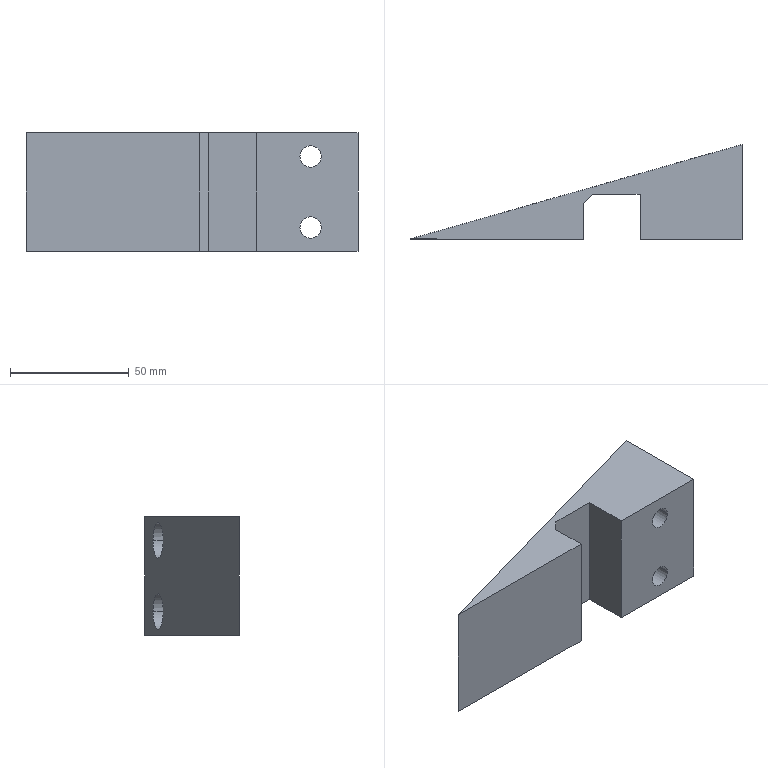Component | SolidWorks | SHYTJ-01-07-07GuideBlock-1 | 1 solid | 20 faces | box 140 x 40 x 50 mm | volume 107982 mm3 | plane 12 | cylinder 8 | commonest cylinder face diameters 15 x4 9 x4
build123d program:
from build123d import *

# Parameters (mm, degrees)
BOSS_EXTRUDE1_DEPTH                               = 50
CUT_EXTRUDE1_DEPTH                                = 154.948
HOLE_SIZE_ACCORDING_TO_TYPE_OF_SOCKET_D           = 9
HOLE_SIZE_ACCORDING_TO_TYPE_OF_SOCKET_CBORE_D     = 15
HOLE_SIZE_ACCORDING_TO_TYPE_OF_SOCKET_CBORE_DEPTH = 29


with BuildPart() as part:
    # Sketch1 → Boss-Extrude1 (new body)
    with BuildSketch(Plane.XY):
        Polygon((0, 0), (0, 40), (140, 0.149), align=None)
    extrude(amount=BOSS_EXTRUDE1_DEPTH)

    # Sketch2 → Cut-Extrude1 (cut, through all)
    with BuildSketch(Plane.XY.offset(50)):
        Polygon((43, 19.046), (63, 19.046), (67, 15.046), (67, 0.04577), (43, 0.04577), align=None)
    extrude(amount=-CUT_EXTRUDE1_DEPTH, mode=Mode.SUBTRACT)

    # Hole Size _according to_ type of socket (through all)
    with Locations(Plane(origin=(-0.04258, 40, 0), x_dir=(-1, -0.001064, 0), z_dir=(-0.001064, 1, 0))):
        with Locations((-20, 10), (-20, 40)):
            CounterBoreHole(HOLE_SIZE_ACCORDING_TO_TYPE_OF_SOCKET_D / 2, HOLE_SIZE_ACCORDING_TO_TYPE_OF_SOCKET_CBORE_D / 2, HOLE_SIZE_ACCORDING_TO_TYPE_OF_SOCKET_CBORE_DEPTH)


solid = part.part

# Placed as in the assembly
solid = solid.moved(Location((-59.116, -175.361, 293.5), (-180, 0, 180)))
STEP:
#1=COLOUR_RGB('',0.7922,0.8196,0.9333);
#2=FILL_AREA_STYLE_COLOUR('',#1);
#3=FILL_AREA_STYLE('',(#2));
#4=SURFACE_STYLE_FILL_AREA(#3);
#5=SURFACE_SIDE_STYLE('',(#4));
#6=SURFACE_STYLE_USAGE(.BOTH.,#5);
#7=PRESENTATION_STYLE_ASSIGNMENT((#6));
#8=CARTESIAN_POINT('',(-3.41,-6.47,11.161));
#9=VERTEX_POINT('',#8);
#10=CARTESIAN_POINT('',(-2.819,-6.47,11.161));
#11=VERTEX_POINT('',#10);
#12=CARTESIAN_POINT('',(-3.114,-6.47,11.161));
#13=DIRECTION('',(0.001064,1.,0.));
#14=DIRECTION('',(1.,-0.001064,0.));
#15=AXIS2_PLACEMENT_3D('',#12,#13,#14);
#16=CIRCLE('',#15,0.2953);
#17=EDGE_CURVE('',#9,#11,#16,.T.);
#18=ORIENTED_EDGE('',*,*,#17,.F.);
#19=CARTESIAN_POINT('',(-3.409,-5.637,11.161));
#20=VERTEX_POINT('',#19);
#21=CARTESIAN_POINT('',(-3.408,-5.328,11.161));
#22=DIRECTION('',(0.001064,1.,0.));
#23=VECTOR('',#22,39.37);
#24=LINE('',#21,#23);
#25=EDGE_CURVE('',#9,#20,#24,.T.);
#26=ORIENTED_EDGE('',*,*,#25,.T.);
#27=CARTESIAN_POINT('',(-2.818,-5.469,11.161));
#28=VERTEX_POINT('',#27);
#29=CARTESIAN_POINT('',(-2.818,-5.469,11.161));
#30=CARTESIAN_POINT('',(-2.818,-5.469,11.752));
#31=CARTESIAN_POINT('',(-3.409,-5.637,11.752));
#32=CARTESIAN_POINT('',(-3.409,-5.637,11.161));
#33=(BOUNDED_CURVE()B_SPLINE_CURVE(3,(#29,#30,#31,#32),.UNSPECIFIED.,.F.,.T.)B_SPLINE_CURVE_WITH_KNOTS((4,4),(0.,3.142),.UNSPECIFIED.)CURVE()GEOMETRIC_REPRESENTATION_ITEM()RATIONAL_B_SPLINE_CURVE((1.,0.3333,0.3333,1.))REPRESENTATION_ITEM(''));
#34=EDGE_CURVE('',#28,#20,#33,.T.);
#35=ORIENTED_EDGE('',*,*,#34,.F.);
#36=CARTESIAN_POINT('',(-2.818,-5.329,11.161));
#37=DIRECTION('',(0.001064,1.,0.));
#38=VECTOR('',#37,39.37);
#39=LINE('',#36,#38);
#40=EDGE_CURVE('',#11,#28,#39,.T.);
#41=ORIENTED_EDGE('',*,*,#40,.F.);
#42=EDGE_LOOP('',(#18,#26,#35,#41));
#43=FACE_OUTER_BOUND('',#42,.T.);
#44=CARTESIAN_POINT('',(-3.113,-5.328,11.161));
#45=DIRECTION('',(0.001064,1.,0.));
#46=DIRECTION('',(1.,-0.001064,0.));
#47=AXIS2_PLACEMENT_3D('',#44,#45,#46);
#48=CYLINDRICAL_SURFACE('',#47,0.2953);
#49=ADVANCED_FACE('',(#43),#48,.F.);
#50=CARTESIAN_POINT('',(-3.292,-6.903,11.161));
#51=VERTEX_POINT('',#50);
#52=CARTESIAN_POINT('',(-2.938,-6.903,11.161));
#53=VERTEX_POINT('',#52);
#54=CARTESIAN_POINT('',(-3.115,-6.903,11.161));
#55=DIRECTION('',(0.001064,1.,0.));
#56=DIRECTION('',(1.,-0.001064,0.));
#57=AXIS2_PLACEMENT_3D('',#54,#55,#56);
#58=CIRCLE('',#57,0.1772);
#59=EDGE_CURVE('',#51,#53,#58,.T.);
#60=ORIENTED_EDGE('',*,*,#59,.F.);
#61=CARTESIAN_POINT('',(-3.292,-6.47,11.161));
#62=VERTEX_POINT('',#61);
#63=CARTESIAN_POINT('',(-3.29,-5.328,11.161));
#64=DIRECTION('',(0.001064,1.,0.));
#65=VECTOR('',#64,39.37);
#66=LINE('',#63,#65);
#67=EDGE_CURVE('',#51,#62,#66,.T.);
#68=ORIENTED_EDGE('',*,*,#67,.T.);
#69=CARTESIAN_POINT('',(-2.937,-6.47,11.161));
#70=VERTEX_POINT('',#69);
#71=CARTESIAN_POINT('',(-3.114,-6.47,11.161));
#72=DIRECTION('',(0.001064,1.,0.));
#73=DIRECTION('',(1.,-0.001064,0.));
#74=AXIS2_PLACEMENT_3D('',#71,#72,#73);
#75=CIRCLE('',#74,0.1772);
#76=EDGE_CURVE('',#62,#70,#75,.T.);
#77=ORIENTED_EDGE('',*,*,#76,.T.);
#78=CARTESIAN_POINT('',(-2.936,-5.329,11.161));
#79=DIRECTION('',(0.001064,1.,0.));
#80=VECTOR('',#79,39.37);
#81=LINE('',#78,#80);
#82=EDGE_CURVE('',#53,#70,#81,.T.);
#83=ORIENTED_EDGE('',*,*,#82,.F.);
#84=EDGE_LOOP('',(#60,#68,#77,#83));
#85=FACE_OUTER_BOUND('',#84,.T.);
#86=CARTESIAN_POINT('',(-3.113,-5.328,11.161));
#87=DIRECTION('',(0.001064,1.,0.));
#88=DIRECTION('',(1.,-0.001064,0.));
#89=AXIS2_PLACEMENT_3D('',#86,#87,#88);
#90=CYLINDRICAL_SURFACE('',#89,0.1772);
#91=ADVANCED_FACE('',(#85),#90,.F.);
#92=CARTESIAN_POINT('',(-3.292,-6.903,9.98));
#93=VERTEX_POINT('',#92);
#94=CARTESIAN_POINT('',(-2.938,-6.903,9.98));
#95=VERTEX_POINT('',#94);
#96=CARTESIAN_POINT('',(-3.115,-6.903,9.98));
#97=DIRECTION('',(0.001064,1.,0.));
#98=DIRECTION('',(1.,-0.001064,0.));
#99=AXIS2_PLACEMENT_3D('',#96,#97,#98);
#100=CIRCLE('',#99,0.1772);
#101=EDGE_CURVE('',#93,#95,#100,.T.);
#102=ORIENTED_EDGE('',*,*,#101,.F.);
#103=CARTESIAN_POINT('',(-3.292,-6.47,9.98));
#104=VERTEX_POINT('',#103);
#105=CARTESIAN_POINT('',(-3.29,-5.328,9.98));
#106=DIRECTION('',(0.001064,1.,0.));
#107=VECTOR('',#106,39.37);
#108=LINE('',#105,#107);
#109=EDGE_CURVE('',#93,#104,#108,.T.);
#110=ORIENTED_EDGE('',*,*,#109,.T.);
#111=CARTESIAN_POINT('',(-2.937,-6.47,9.98));
#112=VERTEX_POINT('',#111);
#113=CARTESIAN_POINT('',(-3.114,-6.47,9.98));
#114=DIRECTION('',(0.001064,1.,0.));
#115=DIRECTION('',(1.,-0.001064,0.));
#116=AXIS2_PLACEMENT_3D('',#113,#114,#115);
#117=CIRCLE('',#116,0.1772);
#118=EDGE_CURVE('',#104,#112,#117,.T.);
#119=ORIENTED_EDGE('',*,*,#118,.T.);
#120=CARTESIAN_POINT('',(-2.936,-5.329,9.98));
#121=DIRECTION('',(0.001064,1.,0.));
#122=VECTOR('',#121,39.37);
#123=LINE('',#120,#122);
#124=EDGE_CURVE('',#95,#112,#123,.T.);
#125=ORIENTED_EDGE('',*,*,#124,.F.);
#126=EDGE_LOOP('',(#102,#110,#119,#125));
#127=FACE_OUTER_BOUND('',#126,.T.);
#128=CARTESIAN_POINT('',(-3.113,-5.328,9.98));
#129=DIRECTION('',(0.001064,1.,0.));
#130=DIRECTION('',(1.,-0.001064,0.));
#131=AXIS2_PLACEMENT_3D('',#128,#129,#130);
#132=CYLINDRICAL_SURFACE('',#131,0.1772);
#133=ADVANCED_FACE('',(#127),#132,.F.);
#134=CARTESIAN_POINT('',(-3.41,-6.47,9.98));
#135=VERTEX_POINT('',#134);
#136=CARTESIAN_POINT('',(-2.819,-6.47,9.98));
#137=VERTEX_POINT('',#136);
#138=CARTESIAN_POINT('',(-3.114,-6.47,9.98));
#139=DIRECTION('',(0.001064,1.,0.));
#140=DIRECTION('',(1.,-0.001064,0.));
#141=AXIS2_PLACEMENT_3D('',#138,#139,#140);
#142=CIRCLE('',#141,0.2953);
#143=EDGE_CURVE('',#135,#137,#142,.T.);
#144=ORIENTED_EDGE('',*,*,#143,.F.);
#145=CARTESIAN_POINT('',(-3.409,-5.637,9.98));
#146=VERTEX_POINT('',#145);
#147=CARTESIAN_POINT('',(-3.408,-5.328,9.98));
#148=DIRECTION('',(0.001064,1.,0.));
#149=VECTOR('',#148,39.37);
#150=LINE('',#147,#149);
#151=EDGE_CURVE('',#135,#146,#150,.T.);
#152=ORIENTED_EDGE('',*,*,#151,.T.);
#153=CARTESIAN_POINT('',(-2.818,-5.469,9.98));
#154=VERTEX_POINT('',#153);
#155=CARTESIAN_POINT('',(-2.818,-5.469,9.98));
#156=CARTESIAN_POINT('',(-2.818,-5.469,10.571));
#157=CARTESIAN_POINT('',(-3.409,-5.637,10.571));
#158=CARTESIAN_POINT('',(-3.409,-5.637,9.98));
#159=(BOUNDED_CURVE()B_SPLINE_CURVE(3,(#155,#156,#157,#158),.UNSPECIFIED.,.F.,.T.)B_SPLINE_CURVE_WITH_KNOTS((4,4),(0.,3.142),.UNSPECIFIED.)CURVE()GEOMETRIC_REPRESENTATION_ITEM()RATIONAL_B_SPLINE_CURVE((1.,0.3333,0.3333,1.))REPRESENTATION_ITEM(''));
#160=EDGE_CURVE('',#154,#146,#159,.T.);
#161=ORIENTED_EDGE('',*,*,#160,.F.);
#162=CARTESIAN_POINT('',(-2.818,-5.329,9.98));
#163=DIRECTION('',(0.001064,1.,0.));
#164=VECTOR('',#163,39.37);
#165=LINE('',#162,#164);
#166=EDGE_CURVE('',#137,#154,#165,.T.);
#167=ORIENTED_EDGE('',*,*,#166,.F.);
#168=EDGE_LOOP('',(#144,#152,#161,#167));
#169=FACE_OUTER_BOUND('',#168,.T.);
#170=CARTESIAN_POINT('',(-3.113,-5.328,9.98));
#171=DIRECTION('',(0.001064,1.,0.));
#172=DIRECTION('',(1.,-0.001064,0.));
#173=AXIS2_PLACEMENT_3D('',#170,#171,#172);
#174=CYLINDRICAL_SURFACE('',#173,0.2953);
#175=ADVANCED_FACE('',(#169),#174,.F.);
#176=CARTESIAN_POINT('',(-4.965,-6.901,9.587));
#177=VERTEX_POINT('',#176);
#178=CARTESIAN_POINT('',(-7.839,-6.898,9.587));
#179=VERTEX_POINT('',#178);
#180=CARTESIAN_POINT('',(-7.839,-6.898,9.587));
#181=DIRECTION('',(-1.,0.001064,0.));
#182=VECTOR('',#181,39.37);
#183=LINE('',#180,#182);
#184=EDGE_CURVE('',#177,#179,#183,.T.);
#185=ORIENTED_EDGE('',*,*,#184,.F.);
#186=CARTESIAN_POINT('',(-4.965,-6.901,11.555));
#187=VERTEX_POINT('',#186);
#188=CARTESIAN_POINT('',(-4.965,-6.901,9.587));
#189=DIRECTION('',(0.,-0.,1.));
#190=VECTOR('',#189,39.37);
#191=LINE('',#188,#190);
#192=EDGE_CURVE('',#177,#187,#191,.T.);
#193=ORIENTED_EDGE('',*,*,#192,.T.);
#194=CARTESIAN_POINT('',(-7.839,-6.898,11.555));
#195=VERTEX_POINT('',#194);
#196=CARTESIAN_POINT('',(-7.839,-6.898,11.555));
#197=DIRECTION('',(-1.,0.001064,0.));
#198=VECTOR('',#197,39.37);
#199=LINE('',#196,#198);
#200=EDGE_CURVE('',#187,#195,#199,.T.);
#201=ORIENTED_EDGE('',*,*,#200,.T.);
#202=CARTESIAN_POINT('',(-7.839,-6.898,9.587));
#203=DIRECTION('',(0.,-0.,1.));
#204=VECTOR('',#203,39.37);
#205=LINE('',#202,#204);
#206=EDGE_CURVE('',#179,#195,#205,.T.);
#207=ORIENTED_EDGE('',*,*,#206,.F.);
#208=EDGE_LOOP('',(#185,#193,#201,#207));
#209=FACE_OUTER_BOUND('',#208,.T.);
#210=CARTESIAN_POINT('',(-7.839,-6.898,9.587));
#211=DIRECTION('',(0.001064,1.,0.));
#212=DIRECTION('',(1.,-0.001064,-0.));
#213=AXIS2_PLACEMENT_3D('',#210,#211,#212);
#214=PLANE('',#213);
#215=ADVANCED_FACE('',(#209),#214,.F.);
#216=CARTESIAN_POINT('',(-3.115,-6.903,11.161));
#217=DIRECTION('',(0.001064,1.,0.));
#218=DIRECTION('',(1.,-0.001064,0.));
#219=AXIS2_PLACEMENT_3D('',#216,#217,#218);
#220=CIRCLE('',#219,0.1772);
#221=EDGE_CURVE('',#53,#51,#220,.T.);
#222=ORIENTED_EDGE('',*,*,#221,.T.);
#223=ORIENTED_EDGE('',*,*,#59,.T.);
#224=EDGE_LOOP('',(#222,#223));
#225=FACE_BOUND('',#224,.T.);
#226=CARTESIAN_POINT('',(-3.115,-6.903,9.98));
#227=DIRECTION('',(0.001064,1.,0.));
#228=DIRECTION('',(1.,-0.001064,0.));
#229=AXIS2_PLACEMENT_3D('',#226,#227,#228);
#230=CIRCLE('',#229,0.1772);
#231=EDGE_CURVE('',#95,#93,#230,.T.);
#232=ORIENTED_EDGE('',*,*,#231,.T.);
#233=ORIENTED_EDGE('',*,*,#101,.T.);
#234=EDGE_LOOP('',(#232,#233));
#235=FACE_BOUND('',#234,.T.);
#236=CARTESIAN_POINT('',(-2.327,-6.904,11.555));
#237=VERTEX_POINT('',#236);
#238=CARTESIAN_POINT('',(-4.02,-6.902,11.555));
#239=VERTEX_POINT('',#238);
#240=CARTESIAN_POINT('',(-7.839,-6.898,11.555));
#241=DIRECTION('',(-1.,0.001064,0.));
#242=VECTOR('',#241,39.37);
#243=LINE('',#240,#242);
#244=EDGE_CURVE('',#237,#239,#243,.T.);
#245=ORIENTED_EDGE('',*,*,#244,.T.);
#246=CARTESIAN_POINT('',(-4.02,-6.902,9.587));
#247=VERTEX_POINT('',#246);
#248=CARTESIAN_POINT('',(-4.02,-6.902,11.555));
#249=DIRECTION('',(-0.,0.,-1.));
#250=VECTOR('',#249,39.37);
#251=LINE('',#248,#250);
#252=EDGE_CURVE('',#239,#247,#251,.T.);
#253=ORIENTED_EDGE('',*,*,#252,.T.);
#254=CARTESIAN_POINT('',(-2.327,-6.904,9.587));
#255=VERTEX_POINT('',#254);
#256=CARTESIAN_POINT('',(-7.839,-6.898,9.587));
#257=DIRECTION('',(-1.,0.001064,0.));
#258=VECTOR('',#257,39.37);
#259=LINE('',#256,#258);
#260=EDGE_CURVE('',#255,#247,#259,.T.);
#261=ORIENTED_EDGE('',*,*,#260,.F.);
#262=CARTESIAN_POINT('',(-2.327,-6.904,9.587));
#263=DIRECTION('',(0.,-0.,1.));
#264=VECTOR('',#263,39.37);
#265=LINE('',#262,#264);
#266=EDGE_CURVE('',#255,#237,#265,.T.);
#267=ORIENTED_EDGE('',*,*,#266,.T.);
#268=EDGE_LOOP('',(#245,#253,#261,#267));
#269=FACE_OUTER_BOUND('',#268,.T.);
#270=CARTESIAN_POINT('',(-7.839,-6.898,9.587));
#271=DIRECTION('',(0.001064,1.,0.));
#272=DIRECTION('',(1.,-0.001064,-0.));
#273=AXIS2_PLACEMENT_3D('',#270,#271,#272);
#274=PLANE('',#273);
#275=ADVANCED_FACE('',(#225,#235,#269),#274,.F.);
#276=ORIENTED_EDGE('',*,*,#34,.T.);
#277=CARTESIAN_POINT('',(-3.409,-5.637,11.161));
#278=CARTESIAN_POINT('',(-3.409,-5.637,10.571));
#279=CARTESIAN_POINT('',(-2.818,-5.469,10.571));
#280=CARTESIAN_POINT('',(-2.818,-5.469,11.161));
#281=(BOUNDED_CURVE()B_SPLINE_CURVE(3,(#277,#278,#279,#280),.UNSPECIFIED.,.F.,.T.)B_SPLINE_CURVE_WITH_KNOTS((4,4),(3.142,6.283),.UNSPECIFIED.)CURVE()GEOMETRIC_REPRESENTATION_ITEM()RATIONAL_B_SPLINE_CURVE((1.,0.3333,0.3333,1.))REPRESENTATION_ITEM(''));
#282=EDGE_CURVE('',#20,#28,#281,.T.);
#283=ORIENTED_EDGE('',*,*,#282,.T.);
#284=EDGE_LOOP('',(#276,#283));
#285=FACE_BOUND('',#284,.T.);
#286=ORIENTED_EDGE('',*,*,#160,.T.);
#287=CARTESIAN_POINT('',(-3.409,-5.637,9.98));
#288=CARTESIAN_POINT('',(-3.409,-5.637,9.39));
#289=CARTESIAN_POINT('',(-2.818,-5.469,9.39));
#290=CARTESIAN_POINT('',(-2.818,-5.469,9.98));
#291=(BOUNDED_CURVE()B_SPLINE_CURVE(3,(#287,#288,#289,#290),.UNSPECIFIED.,.F.,.F.)B_SPLINE_CURVE_WITH_KNOTS((4,4),(3.142,6.283),.UNSPECIFIED.)CURVE()GEOMETRIC_REPRESENTATION_ITEM()RATIONAL_B_SPLINE_CURVE((1.,0.3333,0.3333,1.))REPRESENTATION_ITEM(''));
#292=EDGE_CURVE('',#146,#154,#291,.T.);
#293=ORIENTED_EDGE('',*,*,#292,.T.);
#294=EDGE_LOOP('',(#286,#293));
#295=FACE_BOUND('',#294,.T.);
#296=CARTESIAN_POINT('',(-2.327,-5.329,11.555));
#297=VERTEX_POINT('',#296);
#298=CARTESIAN_POINT('',(-2.327,-5.329,11.555));
#299=DIRECTION('',(0.9618,0.2738,-0.));
#300=VECTOR('',#299,39.37);
#301=LINE('',#298,#300);
#302=EDGE_CURVE('',#195,#297,#301,.T.);
#303=ORIENTED_EDGE('',*,*,#302,.T.);
#304=CARTESIAN_POINT('',(-2.327,-5.329,9.587));
#305=VERTEX_POINT('',#304);
#306=CARTESIAN_POINT('',(-2.327,-5.329,9.587));
#307=DIRECTION('',(0.,-0.,1.));
#308=VECTOR('',#307,39.37);
#309=LINE('',#306,#308);
#310=EDGE_CURVE('',#305,#297,#309,.T.);
#311=ORIENTED_EDGE('',*,*,#310,.F.);
#312=CARTESIAN_POINT('',(-2.327,-5.329,9.587));
#313=DIRECTION('',(0.9618,0.2738,-0.));
#314=VECTOR('',#313,39.37);
#315=LINE('',#312,#314);
#316=EDGE_CURVE('',#179,#305,#315,.T.);
#317=ORIENTED_EDGE('',*,*,#316,.F.);
#318=ORIENTED_EDGE('',*,*,#206,.T.);
#319=EDGE_LOOP('',(#303,#311,#317,#318));
#320=FACE_OUTER_BOUND('',#319,.T.);
#321=CARTESIAN_POINT('',(-2.327,-5.329,9.587));
#322=DIRECTION('',(0.2738,-0.9618,-0.));
#323=DIRECTION('',(-0.9618,-0.2738,0.));
#324=AXIS2_PLACEMENT_3D('',#321,#322,#323);
#325=PLANE('',#324);
#326=ADVANCED_FACE('',(#285,#295,#320),#325,.F.);
#327=CARTESIAN_POINT('',(-2.327,-6.904,11.555));
#328=DIRECTION('',(0.,-1.,-0.));
#329=VECTOR('',#328,39.37);
#330=LINE('',#327,#329);
#331=EDGE_CURVE('',#297,#237,#330,.T.);
#332=ORIENTED_EDGE('',*,*,#331,.T.);
#333=ORIENTED_EDGE('',*,*,#266,.F.);
#334=CARTESIAN_POINT('',(-2.327,-6.904,9.587));
#335=DIRECTION('',(0.,-1.,-0.));
#336=VECTOR('',#335,39.37);
#337=LINE('',#334,#336);
#338=EDGE_CURVE('',#305,#255,#337,.T.);
#339=ORIENTED_EDGE('',*,*,#338,.F.);
#340=ORIENTED_EDGE('',*,*,#310,.T.);
#341=EDGE_LOOP('',(#332,#333,#339,#340));
#342=FACE_OUTER_BOUND('',#341,.T.);
#343=CARTESIAN_POINT('',(-2.327,-6.904,9.587));
#344=DIRECTION('',(-1.,-0.,0.));
#345=DIRECTION('',(0.,-0.,1.));
#346=AXIS2_PLACEMENT_3D('',#343,#344,#345);
#347=PLANE('',#346);
#348=ADVANCED_FACE('',(#342),#347,.F.);
#349=ORIENTED_EDGE('',*,*,#260,.T.);
#350=CARTESIAN_POINT('',(-4.02,-6.154,9.587));
#351=VERTEX_POINT('',#350);
#352=CARTESIAN_POINT('',(-4.02,-6.154,9.587));
#353=DIRECTION('',(0.,-1.,-0.));
#354=VECTOR('',#353,39.37);
#355=LINE('',#352,#354);
#356=EDGE_CURVE('',#351,#247,#355,.T.);
#357=ORIENTED_EDGE('',*,*,#356,.F.);
#358=CARTESIAN_POINT('',(-4.808,-6.154,9.587));
#359=VERTEX_POINT('',#358);
#360=CARTESIAN_POINT('',(-4.02,-6.154,9.587));
#361=DIRECTION('',(1.,-0.,-0.));
#362=VECTOR('',#361,39.37);
#363=LINE('',#360,#362);
#364=EDGE_CURVE('',#359,#351,#363,.T.);
#365=ORIENTED_EDGE('',*,*,#364,.F.);
#366=CARTESIAN_POINT('',(-4.965,-6.312,9.587));
#367=VERTEX_POINT('',#366);
#368=CARTESIAN_POINT('',(-4.808,-6.154,9.587));
#369=DIRECTION('',(0.7071,0.7071,-0.));
#370=VECTOR('',#369,39.37);
#371=LINE('',#368,#370);
#372=EDGE_CURVE('',#367,#359,#371,.T.);
#373=ORIENTED_EDGE('',*,*,#372,.F.);
#374=CARTESIAN_POINT('',(-4.965,-6.312,9.587));
#375=DIRECTION('',(-0.,1.,0.));
#376=VECTOR('',#375,39.37);
#377=LINE('',#374,#376);
#378=EDGE_CURVE('',#177,#367,#377,.T.);
#379=ORIENTED_EDGE('',*,*,#378,.F.);
#380=ORIENTED_EDGE('',*,*,#184,.T.);
#381=ORIENTED_EDGE('',*,*,#316,.T.);
#382=ORIENTED_EDGE('',*,*,#338,.T.);
#383=EDGE_LOOP('',(#349,#357,#365,#373,#379,#380,#381,#382));
#384=FACE_OUTER_BOUND('',#383,.T.);
#385=CARTESIAN_POINT('',(-2.327,-6.904,9.587));
#386=DIRECTION('',(0.,-0.,1.));
#387=DIRECTION('',(1.,0.,-0.));
#388=AXIS2_PLACEMENT_3D('',#385,#386,#387);
#389=PLANE('',#388);
#390=ADVANCED_FACE('',(#384),#389,.F.);
#391=CARTESIAN_POINT('',(-4.02,-6.154,11.555));
#392=VERTEX_POINT('',#391);
#393=CARTESIAN_POINT('',(-4.02,-6.154,11.555));
#394=DIRECTION('',(0.,-1.,-0.));
#395=VECTOR('',#394,39.37);
#396=LINE('',#393,#395);
#397=EDGE_CURVE('',#392,#239,#396,.T.);
#398=ORIENTED_EDGE('',*,*,#397,.T.);
#399=ORIENTED_EDGE('',*,*,#244,.F.);
#400=ORIENTED_EDGE('',*,*,#331,.F.);
#401=ORIENTED_EDGE('',*,*,#302,.F.);
#402=ORIENTED_EDGE('',*,*,#200,.F.);
#403=CARTESIAN_POINT('',(-4.965,-6.312,11.555));
#404=VERTEX_POINT('',#403);
#405=CARTESIAN_POINT('',(-4.965,-6.904,11.555));
#406=DIRECTION('',(0.,-1.,-0.));
#407=VECTOR('',#406,39.37);
#408=LINE('',#405,#407);
#409=EDGE_CURVE('',#404,#187,#408,.T.);
#410=ORIENTED_EDGE('',*,*,#409,.F.);
#411=CARTESIAN_POINT('',(-4.808,-6.154,11.555));
#412=VERTEX_POINT('',#411);
#413=CARTESIAN_POINT('',(-4.808,-6.154,11.555));
#414=DIRECTION('',(0.7071,0.7071,-0.));
#415=VECTOR('',#414,39.37);
#416=LINE('',#413,#415);
#417=EDGE_CURVE('',#404,#412,#416,.T.);
#418=ORIENTED_EDGE('',*,*,#417,.T.);
#419=CARTESIAN_POINT('',(-4.02,-6.154,11.555));
#420=DIRECTION('',(1.,-0.,-0.));
#421=VECTOR('',#420,39.37);
#422=LINE('',#419,#421);
#423=EDGE_CURVE('',#412,#392,#422,.T.);
#424=ORIENTED_EDGE('',*,*,#423,.T.);
#425=EDGE_LOOP('',(#398,#399,#400,#401,#402,#410,#418,#424));
#426=FACE_OUTER_BOUND('',#425,.T.);
#427=CARTESIAN_POINT('',(-2.327,-6.904,11.555));
#428=DIRECTION('',(0.,-0.,1.));
#429=DIRECTION('',(1.,0.,-0.));
#430=AXIS2_PLACEMENT_3D('',#427,#428,#429);
#431=PLANE('',#430);
#432=ADVANCED_FACE('',(#426),#431,.T.);
#433=ORIENTED_EDGE('',*,*,#378,.T.);
#434=CARTESIAN_POINT('',(-4.965,-6.312,11.555));
#435=DIRECTION('',(-0.,0.,-1.));
#436=VECTOR('',#435,39.37);
#437=LINE('',#434,#436);
#438=EDGE_CURVE('',#404,#367,#437,.T.);
#439=ORIENTED_EDGE('',*,*,#438,.F.);
#440=ORIENTED_EDGE('',*,*,#409,.T.);
#441=ORIENTED_EDGE('',*,*,#192,.F.);
#442=EDGE_LOOP('',(#433,#439,#440,#441));
#443=FACE_OUTER_BOUND('',#442,.T.);
#444=CARTESIAN_POINT('',(-4.965,-6.312,11.555));
#445=DIRECTION('',(-1.,-0.,0.));
#446=DIRECTION('',(0.,-0.,1.));
#447=AXIS2_PLACEMENT_3D('',#444,#445,#446);
#448=PLANE('',#447);
#449=ADVANCED_FACE('',(#443),#448,.F.);
#450=ORIENTED_EDGE('',*,*,#356,.T.);
#451=ORIENTED_EDGE('',*,*,#252,.F.);
#452=ORIENTED_EDGE('',*,*,#397,.F.);
#453=CARTESIAN_POINT('',(-4.02,-6.154,11.555));
#454=DIRECTION('',(-0.,0.,-1.));
#455=VECTOR('',#454,39.37);
#456=LINE('',#453,#455);
#457=EDGE_CURVE('',#392,#351,#456,.T.);
#458=ORIENTED_EDGE('',*,*,#457,.T.);
#459=EDGE_LOOP('',(#450,#451,#452,#458));
#460=FACE_OUTER_BOUND('',#459,.T.);
#461=CARTESIAN_POINT('',(-4.02,-6.154,11.555));
#462=DIRECTION('',(1.,0.,-0.));
#463=DIRECTION('',(-0.,0.,-1.));
#464=AXIS2_PLACEMENT_3D('',#461,#462,#463);
#465=PLANE('',#464);
#466=ADVANCED_FACE('',(#460),#465,.F.);
#467=ORIENTED_EDGE('',*,*,#364,.T.);
#468=ORIENTED_EDGE('',*,*,#457,.F.);
#469=ORIENTED_EDGE('',*,*,#423,.F.);
#470=CARTESIAN_POINT('',(-4.808,-6.154,11.555));
#471=DIRECTION('',(-0.,0.,-1.));
#472=VECTOR('',#471,39.37);
#473=LINE('',#470,#472);
#474=EDGE_CURVE('',#412,#359,#473,.T.);
#475=ORIENTED_EDGE('',*,*,#474,.T.);
#476=EDGE_LOOP('',(#467,#468,#469,#475));
#477=FACE_OUTER_BOUND('',#476,.T.);
#478=CARTESIAN_POINT('',(-4.02,-6.154,11.555));
#479=DIRECTION('',(0.,1.,0.));
#480=DIRECTION('',(1.,-0.,-0.));
#481=AXIS2_PLACEMENT_3D('',#478,#479,#480);
#482=PLANE('',#481);
#483=ADVANCED_FACE('',(#477),#482,.F.);
#484=ORIENTED_EDGE('',*,*,#372,.T.);
#485=ORIENTED_EDGE('',*,*,#474,.F.);
#486=ORIENTED_EDGE('',*,*,#417,.F.);
#487=ORIENTED_EDGE('',*,*,#438,.T.);
#488=EDGE_LOOP('',(#484,#485,#486,#487));
#489=FACE_OUTER_BOUND('',#488,.T.);
#490=CARTESIAN_POINT('',(-4.808,-6.154,11.555));
#491=DIRECTION('',(-0.7071,0.7071,0.));
#492=DIRECTION('',(0.7071,0.7071,-0.));
#493=AXIS2_PLACEMENT_3D('',#490,#491,#492);
#494=PLANE('',#493);
#495=ADVANCED_FACE('',(#489),#494,.F.);
#496=ORIENTED_EDGE('',*,*,#151,.F.);
#497=CARTESIAN_POINT('',(-3.114,-6.47,9.98));
#498=DIRECTION('',(0.001064,1.,0.));
#499=DIRECTION('',(1.,-0.001064,0.));
#500=AXIS2_PLACEMENT_3D('',#497,#498,#499);
#501=CIRCLE('',#500,0.2953);
#502=EDGE_CURVE('',#137,#135,#501,.T.);
#503=ORIENTED_EDGE('',*,*,#502,.F.);
#504=ORIENTED_EDGE('',*,*,#166,.T.);
#505=ORIENTED_EDGE('',*,*,#292,.F.);
#506=EDGE_LOOP('',(#496,#503,#504,#505));
#507=FACE_OUTER_BOUND('',#506,.T.);
#508=CARTESIAN_POINT('',(-3.113,-5.328,9.98));
#509=DIRECTION('',(0.001064,1.,0.));
#510=DIRECTION('',(1.,-0.001064,0.));
#511=AXIS2_PLACEMENT_3D('',#508,#509,#510);
#512=CYLINDRICAL_SURFACE('',#511,0.2953);
#513=ADVANCED_FACE('',(#507),#512,.F.);
#514=ORIENTED_EDGE('',*,*,#109,.F.);
#515=ORIENTED_EDGE('',*,*,#231,.F.);
#516=ORIENTED_EDGE('',*,*,#124,.T.);
#517=CARTESIAN_POINT('',(-3.114,-6.47,9.98));
#518=DIRECTION('',(0.001064,1.,0.));
#519=DIRECTION('',(1.,-0.001064,0.));
#520=AXIS2_PLACEMENT_3D('',#517,#518,#519);
#521=CIRCLE('',#520,0.1772);
#522=EDGE_CURVE('',#112,#104,#521,.T.);
#523=ORIENTED_EDGE('',*,*,#522,.T.);
#524=EDGE_LOOP('',(#514,#515,#516,#523));
#525=FACE_OUTER_BOUND('',#524,.T.);
#526=CARTESIAN_POINT('',(-3.113,-5.328,9.98));
#527=DIRECTION('',(0.001064,1.,0.));
#528=DIRECTION('',(1.,-0.001064,0.));
#529=AXIS2_PLACEMENT_3D('',#526,#527,#528);
#530=CYLINDRICAL_SURFACE('',#529,0.1772);
#531=ADVANCED_FACE('',(#525),#530,.F.);
#532=ORIENTED_EDGE('',*,*,#522,.F.);
#533=ORIENTED_EDGE('',*,*,#118,.F.);
#534=EDGE_LOOP('',(#532,#533));
#535=FACE_BOUND('',#534,.T.);
#536=ORIENTED_EDGE('',*,*,#502,.T.);
#537=ORIENTED_EDGE('',*,*,#143,.T.);
#538=EDGE_LOOP('',(#536,#537));
#539=FACE_OUTER_BOUND('',#538,.T.);
#540=CARTESIAN_POINT('',(-3.114,-6.47,9.803));
#541=DIRECTION('',(-0.001064,-1.,-0.));
#542=DIRECTION('',(-1.,0.001064,0.));
#543=AXIS2_PLACEMENT_3D('',#540,#541,#542);
#544=PLANE('',#543);
#545=ADVANCED_FACE('',(#535,#539),#544,.F.);
#546=ORIENTED_EDGE('',*,*,#67,.F.);
#547=ORIENTED_EDGE('',*,*,#221,.F.);
#548=ORIENTED_EDGE('',*,*,#82,.T.);
#549=CARTESIAN_POINT('',(-3.114,-6.47,11.161));
#550=DIRECTION('',(0.001064,1.,0.));
#551=DIRECTION('',(1.,-0.001064,0.));
#552=AXIS2_PLACEMENT_3D('',#549,#550,#551);
#553=CIRCLE('',#552,0.1772);
#554=EDGE_CURVE('',#70,#62,#553,.T.);
#555=ORIENTED_EDGE('',*,*,#554,.T.);
#556=EDGE_LOOP('',(#546,#547,#548,#555));
#557=FACE_OUTER_BOUND('',#556,.T.);
#558=CARTESIAN_POINT('',(-3.113,-5.328,11.161));
#559=DIRECTION('',(0.001064,1.,0.));
#560=DIRECTION('',(1.,-0.001064,0.));
#561=AXIS2_PLACEMENT_3D('',#558,#559,#560);
#562=CYLINDRICAL_SURFACE('',#561,0.1772);
#563=ADVANCED_FACE('',(#557),#562,.F.);
#564=ORIENTED_EDGE('',*,*,#25,.F.);
#565=CARTESIAN_POINT('',(-3.114,-6.47,11.161));
#566=DIRECTION('',(0.001064,1.,0.));
#567=DIRECTION('',(1.,-0.001064,0.));
#568=AXIS2_PLACEMENT_3D('',#565,#566,#567);
#569=CIRCLE('',#568,0.2953);
#570=EDGE_CURVE('',#11,#9,#569,.T.);
#571=ORIENTED_EDGE('',*,*,#570,.F.);
#572=ORIENTED_EDGE('',*,*,#40,.T.);
#573=ORIENTED_EDGE('',*,*,#282,.F.);
#574=EDGE_LOOP('',(#564,#571,#572,#573));
#575=FACE_OUTER_BOUND('',#574,.T.);
#576=CARTESIAN_POINT('',(-3.113,-5.328,11.161));
#577=DIRECTION('',(0.001064,1.,0.));
#578=DIRECTION('',(1.,-0.001064,0.));
#579=AXIS2_PLACEMENT_3D('',#576,#577,#578);
#580=CYLINDRICAL_SURFACE('',#579,0.2953);
#581=ADVANCED_FACE('',(#575),#580,.F.);
#582=ORIENTED_EDGE('',*,*,#554,.F.);
#583=ORIENTED_EDGE('',*,*,#76,.F.);
#584=EDGE_LOOP('',(#582,#583));
#585=FACE_BOUND('',#584,.T.);
#586=ORIENTED_EDGE('',*,*,#570,.T.);
#587=ORIENTED_EDGE('',*,*,#17,.T.);
#588=EDGE_LOOP('',(#586,#587));
#589=FACE_OUTER_BOUND('',#588,.T.);
#590=CARTESIAN_POINT('',(-3.114,-6.47,10.984));
#591=DIRECTION('',(-0.001064,-1.,-0.));
#592=DIRECTION('',(-1.,0.001064,0.));
#593=AXIS2_PLACEMENT_3D('',#590,#591,#592);
#594=PLANE('',#593);
#595=ADVANCED_FACE('',(#585,#589),#594,.F.);
#596=CLOSED_SHELL('',(#49,#91,#133,#175,#215,#275,#326,#348,#390,#432,#449,#466,#483,#495,#513,#531,#545,#563,#581,#595));
#597=MANIFOLD_SOLID_BREP('',#596);
#598=STYLED_ITEM('',(#7),#597);
#599=PRESENTATION_LAYER_ASSIGNMENT('','',(#598));
#600=CARTESIAN_POINT('',(0.,0.,0.));
#601=DIRECTION('',(0.,0.,1.));
#602=DIRECTION('',(1.,0.,0.));
#603=AXIS2_PLACEMENT_3D('',#600,#601,#602);
#604=(LENGTH_UNIT()NAMED_UNIT(*)SI_UNIT($,.METRE.));
#605=LENGTH_MEASURE_WITH_UNIT(LENGTH_MEASURE(0.0254),#604);
#606=DIMENSIONAL_EXPONENTS(1.,0.,0.,0.,0.,0.,0.);
#607=(CONVERSION_BASED_UNIT('',#605)LENGTH_UNIT()NAMED_UNIT(#606));
#608=UNCERTAINTY_MEASURE_WITH_UNIT(LENGTH_MEASURE(0.00001),#607,'','');
#609=(NAMED_UNIT(*)PLANE_ANGLE_UNIT()SI_UNIT($,.RADIAN.));
#610=(NAMED_UNIT(*)SI_UNIT($,.STERADIAN.)SOLID_ANGLE_UNIT());
#611=(GEOMETRIC_REPRESENTATION_CONTEXT(3)GLOBAL_UNCERTAINTY_ASSIGNED_CONTEXT((#608))GLOBAL_UNIT_ASSIGNED_CONTEXT((#607,#609,#610))REPRESENTATION_CONTEXT('',''));
#612=ADVANCED_BREP_SHAPE_REPRESENTATION('',(#597,#603),#611);
#613=(LENGTH_UNIT()NAMED_UNIT(*)SI_UNIT($,.METRE.));
#614=LENGTH_MEASURE_WITH_UNIT(LENGTH_MEASURE(0.0254),#613);
#615=DIMENSIONAL_EXPONENTS(1.,0.,0.,0.,0.,0.,0.);
#616=(CONVERSION_BASED_UNIT('',#614)LENGTH_UNIT()NAMED_UNIT(#615));
#617=UNCERTAINTY_MEASURE_WITH_UNIT(LENGTH_MEASURE(0.00001),#616,'','');
#618=(NAMED_UNIT(*)PLANE_ANGLE_UNIT()SI_UNIT($,.RADIAN.));
#619=(NAMED_UNIT(*)SI_UNIT($,.STERADIAN.)SOLID_ANGLE_UNIT());
#620=(GEOMETRIC_REPRESENTATION_CONTEXT(3)GLOBAL_UNCERTAINTY_ASSIGNED_CONTEXT((#617))GLOBAL_UNIT_ASSIGNED_CONTEXT((#616,#618,#619))REPRESENTATION_CONTEXT('',''));
#621=MECHANICAL_DESIGN_GEOMETRIC_PRESENTATION_REPRESENTATION('',(#598),#620);